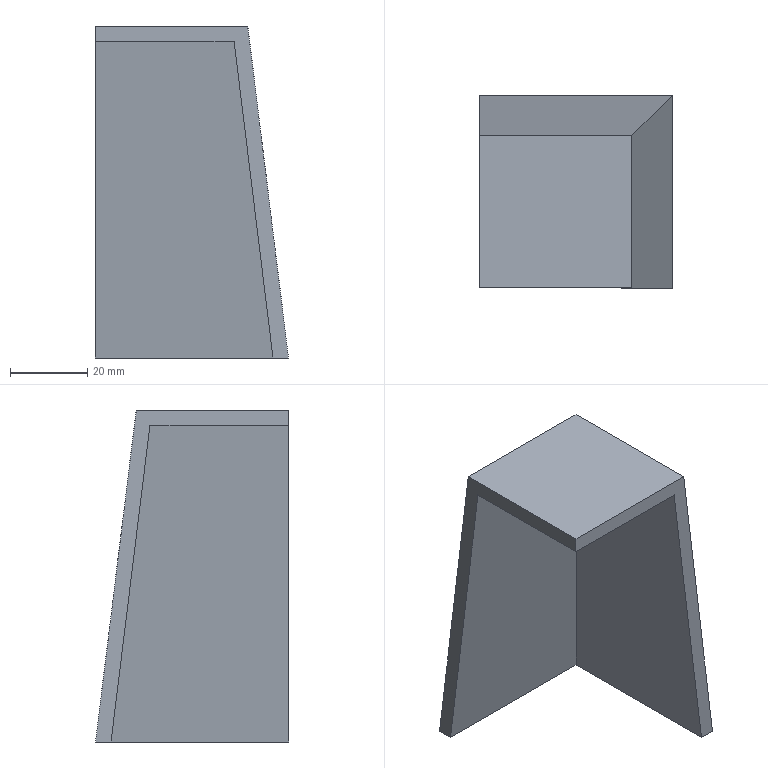Component | NX | STAND_2 | 1 solid | 9 faces | box 50 x 50 x 86 mm | volume 34687 mm3 | plane 9
STEP:
#1=CARTESIAN_POINT('',(0.,0.,0.));
#2=DIRECTION('',(0.,0.,1.));
#3=DIRECTION('',(1.,0.,0.));
#4=AXIS2_PLACEMENT_3D('',#1,#2,#3);
#5=CARTESIAN_POINT('',(223.059,445.97,-786.));
#6=VERTEX_POINT('',#5);
#7=CARTESIAN_POINT('',(223.059,450.,-786.));
#8=VERTEX_POINT('',#7);
#9=CARTESIAN_POINT('',(223.059,400.,-786.));
#10=DIRECTION('',(0.,1.,0.));
#11=VECTOR('',#10,1.);
#12=LINE('',#9,#11);
#13=CARTESIAN_POINT('',(223.059,400.,-770.));
#14=DIRECTION('',(-1.,0.,0.));
#15=DIRECTION('',(0.,0.,-1.));
#16=AXIS2_PLACEMENT_3D('',#13,#14,#15);
#17=PLANE('',#16);
#18=CARTESIAN_POINT('',(16.,0.));
#19=DIRECTION('',(0.,-1.));
#20=VECTOR('',#19,1.);
#21=LINE('',#18,#20);
#22=(GEOMETRIC_REPRESENTATION_CONTEXT(2)PARAMETRIC_REPRESENTATION_CONTEXT()REPRESENTATION_CONTEXT('',''));
#23=DEFINITIONAL_REPRESENTATION('',(#21),#22);
#24=PCURVE('',#17,#23);
#25=CARTESIAN_POINT('',(273.059,400.,-786.));
#26=DIRECTION('',(0.,0.,-1.));
#27=DIRECTION('',(1.,0.,0.));
#28=AXIS2_PLACEMENT_3D('',#25,#26,#27);
#29=PLANE('',#28);
#30=CARTESIAN_POINT('',(-50.,0.));
#31=DIRECTION('',(0.,-1.));
#32=VECTOR('',#31,1.);
#33=LINE('',#30,#32);
#34=(GEOMETRIC_REPRESENTATION_CONTEXT(2)PARAMETRIC_REPRESENTATION_CONTEXT()REPRESENTATION_CONTEXT('',''));
#35=DEFINITIONAL_REPRESENTATION('',(#33),#34);
#36=PCURVE('',#29,#35);
#37=SURFACE_CURVE('',#12,(#24,#36),.PCURVE_S1.);
#38=EDGE_CURVE('',#6,#8,#37,.T.);
#39=ORIENTED_EDGE('',*,*,#38,.F.);
#40=CARTESIAN_POINT('',(223.059,435.902,-704.));
#41=VERTEX_POINT('',#40);
#42=CARTESIAN_POINT('',(223.059,446.03,-786.487));
#43=DIRECTION('',(0.,-0.1219,0.9925));
#44=VECTOR('',#43,1.);
#45=LINE('',#42,#44);
#46=CARTESIAN_POINT('',(16.487,-46.03));
#47=DIRECTION('',(-0.9925,0.1219));
#48=VECTOR('',#47,1.);
#49=LINE('',#46,#48);
#50=(GEOMETRIC_REPRESENTATION_CONTEXT(2)PARAMETRIC_REPRESENTATION_CONTEXT()REPRESENTATION_CONTEXT('',''));
#51=DEFINITIONAL_REPRESENTATION('',(#49),#50);
#52=PCURVE('',#17,#51);
#53=CARTESIAN_POINT('',(248.059,446.03,-786.487));
#54=DIRECTION('',(0.,-0.9925,-0.1219));
#55=DIRECTION('',(0.,-0.1219,0.9925));
#56=AXIS2_PLACEMENT_3D('',#53,#54,#55);
#57=PLANE('',#56);
#58=CARTESIAN_POINT('',(0.,25.));
#59=DIRECTION('',(1.,0.));
#60=VECTOR('',#59,1.);
#61=LINE('',#58,#60);
#62=(GEOMETRIC_REPRESENTATION_CONTEXT(2)PARAMETRIC_REPRESENTATION_CONTEXT()REPRESENTATION_CONTEXT('',''));
#63=DEFINITIONAL_REPRESENTATION('',(#61),#62);
#64=PCURVE('',#57,#63);
#65=SURFACE_CURVE('',#45,(#52,#64),.PCURVE_S1.);
#66=EDGE_CURVE('',#6,#41,#65,.T.);
#67=ORIENTED_EDGE('',*,*,#66,.T.);
#68=CARTESIAN_POINT('',(223.059,400.,-704.));
#69=VERTEX_POINT('',#68);
#70=CARTESIAN_POINT('',(223.059,400.,-704.));
#71=DIRECTION('',(0.,1.,0.));
#72=VECTOR('',#71,1.);
#73=LINE('',#70,#72);
#74=CARTESIAN_POINT('',(-66.,0.));
#75=DIRECTION('',(0.,-1.));
#76=VECTOR('',#75,1.);
#77=LINE('',#74,#76);
#78=(GEOMETRIC_REPRESENTATION_CONTEXT(2)PARAMETRIC_REPRESENTATION_CONTEXT()REPRESENTATION_CONTEXT('',''));
#79=DEFINITIONAL_REPRESENTATION('',(#77),#78);
#80=PCURVE('',#17,#79);
#81=CARTESIAN_POINT('',(223.059,400.,-704.));
#82=DIRECTION('',(0.,0.,1.));
#83=DIRECTION('',(-1.,0.,0.));
#84=AXIS2_PLACEMENT_3D('',#81,#82,#83);
#85=PLANE('',#84);
#86=CARTESIAN_POINT('',(0.,0.));
#87=DIRECTION('',(0.,-1.));
#88=VECTOR('',#87,1.);
#89=LINE('',#86,#88);
#90=(GEOMETRIC_REPRESENTATION_CONTEXT(2)PARAMETRIC_REPRESENTATION_CONTEXT()REPRESENTATION_CONTEXT('',''));
#91=DEFINITIONAL_REPRESENTATION('',(#89),#90);
#92=PCURVE('',#85,#91);
#93=SURFACE_CURVE('',#73,(#80,#92),.PCURVE_S1.);
#94=EDGE_CURVE('',#69,#41,#93,.T.);
#95=ORIENTED_EDGE('',*,*,#94,.F.);
#96=CARTESIAN_POINT('',(223.059,400.,-700.));
#97=VERTEX_POINT('',#96);
#98=CARTESIAN_POINT('',(223.059,400.,-770.));
#99=DIRECTION('',(0.,0.,1.));
#100=VECTOR('',#99,1.);
#101=LINE('',#98,#100);
#102=CARTESIAN_POINT('',(0.,0.));
#103=DIRECTION('',(-1.,0.));
#104=VECTOR('',#103,1.);
#105=LINE('',#102,#104);
#106=(GEOMETRIC_REPRESENTATION_CONTEXT(2)PARAMETRIC_REPRESENTATION_CONTEXT()REPRESENTATION_CONTEXT('',''));
#107=DEFINITIONAL_REPRESENTATION('',(#105),#106);
#108=PCURVE('',#17,#107);
#109=CARTESIAN_POINT('',(0.,400.,0.));
#110=DIRECTION('',(0.,1.,0.));
#111=DIRECTION('',(0.,0.,-1.));
#112=AXIS2_PLACEMENT_3D('',#109,#110,#111);
#113=PLANE('',#112);
#114=CARTESIAN_POINT('',(770.,-223.059));
#115=DIRECTION('',(-1.,0.));
#116=VECTOR('',#115,1.);
#117=LINE('',#114,#116);
#118=(GEOMETRIC_REPRESENTATION_CONTEXT(2)PARAMETRIC_REPRESENTATION_CONTEXT()REPRESENTATION_CONTEXT('',''));
#119=DEFINITIONAL_REPRESENTATION('',(#117),#118);
#120=PCURVE('',#113,#119);
#121=SURFACE_CURVE('',#101,(#108,#120),.PCURVE_S1.);
#122=EDGE_CURVE('',#69,#97,#121,.T.);
#123=ORIENTED_EDGE('',*,*,#122,.T.);
#124=CARTESIAN_POINT('',(223.059,439.441,-700.));
#125=VERTEX_POINT('',#124);
#126=CARTESIAN_POINT('',(223.059,400.,-700.));
#127=DIRECTION('',(0.,1.,0.));
#128=VECTOR('',#127,1.);
#129=LINE('',#126,#128);
#130=CARTESIAN_POINT('',(-70.,0.));
#131=DIRECTION('',(0.,-1.));
#132=VECTOR('',#131,1.);
#133=LINE('',#130,#132);
#134=(GEOMETRIC_REPRESENTATION_CONTEXT(2)PARAMETRIC_REPRESENTATION_CONTEXT()REPRESENTATION_CONTEXT('',''));
#135=DEFINITIONAL_REPRESENTATION('',(#133),#134);
#136=PCURVE('',#17,#135);
#137=CARTESIAN_POINT('',(223.059,400.,-700.));
#138=DIRECTION('',(0.,0.,1.));
#139=DIRECTION('',(-1.,0.,0.));
#140=AXIS2_PLACEMENT_3D('',#137,#138,#139);
#141=PLANE('',#140);
#142=CARTESIAN_POINT('',(0.,0.));
#143=DIRECTION('',(0.,-1.));
#144=VECTOR('',#143,1.);
#145=LINE('',#142,#144);
#146=(GEOMETRIC_REPRESENTATION_CONTEXT(2)PARAMETRIC_REPRESENTATION_CONTEXT()REPRESENTATION_CONTEXT('',''));
#147=DEFINITIONAL_REPRESENTATION('',(#145),#146);
#148=PCURVE('',#141,#147);
#149=SURFACE_CURVE('',#129,(#136,#148),.PCURVE_S1.);
#150=EDGE_CURVE('',#97,#125,#149,.T.);
#151=ORIENTED_EDGE('',*,*,#150,.T.);
#152=CARTESIAN_POINT('',(223.059,450.,-786.));
#153=DIRECTION('',(0.,-0.1219,0.9925));
#154=VECTOR('',#153,1.);
#155=LINE('',#152,#154);
#156=CARTESIAN_POINT('',(16.,-50.));
#157=DIRECTION('',(-0.9925,0.1219));
#158=VECTOR('',#157,1.);
#159=LINE('',#156,#158);
#160=(GEOMETRIC_REPRESENTATION_CONTEXT(2)PARAMETRIC_REPRESENTATION_CONTEXT()REPRESENTATION_CONTEXT('',''));
#161=DEFINITIONAL_REPRESENTATION('',(#159),#160);
#162=PCURVE('',#17,#161);
#163=CARTESIAN_POINT('',(248.059,450.,-786.));
#164=DIRECTION('',(0.,-0.9925,-0.1219));
#165=DIRECTION('',(0.,-0.1219,0.9925));
#166=AXIS2_PLACEMENT_3D('',#163,#164,#165);
#167=PLANE('',#166);
#168=CARTESIAN_POINT('',(0.,25.));
#169=DIRECTION('',(1.,0.));
#170=VECTOR('',#169,1.);
#171=LINE('',#168,#170);
#172=(GEOMETRIC_REPRESENTATION_CONTEXT(2)PARAMETRIC_REPRESENTATION_CONTEXT()REPRESENTATION_CONTEXT('',''));
#173=DEFINITIONAL_REPRESENTATION('',(#171),#172);
#174=PCURVE('',#167,#173);
#175=SURFACE_CURVE('',#155,(#162,#174),.PCURVE_S1.);
#176=EDGE_CURVE('',#8,#125,#175,.T.);
#177=ORIENTED_EDGE('',*,*,#176,.F.);
#178=EDGE_LOOP('',(#39,#67,#95,#123,#151,#177));
#179=FACE_BOUND('',#178,.T.);
#180=ADVANCED_FACE('',(#179),#17,.T.);
#181=CARTESIAN_POINT('',(269.029,400.,-786.));
#182=VERTEX_POINT('',#181);
#183=CARTESIAN_POINT('',(269.029,445.97,-786.));
#184=VERTEX_POINT('',#183);
#185=CARTESIAN_POINT('',(269.029,425.,-786.));
#186=DIRECTION('',(0.,1.,0.));
#187=VECTOR('',#186,1.);
#188=LINE('',#185,#187);
#189=CARTESIAN_POINT('',(-4.03,-25.));
#190=DIRECTION('',(0.,-1.));
#191=VECTOR('',#190,1.);
#192=LINE('',#189,#191);
#193=(GEOMETRIC_REPRESENTATION_CONTEXT(2)PARAMETRIC_REPRESENTATION_CONTEXT()REPRESENTATION_CONTEXT('',''));
#194=DEFINITIONAL_REPRESENTATION('',(#192),#193);
#195=PCURVE('',#29,#194);
#196=CARTESIAN_POINT('',(269.089,425.,-786.487));
#197=DIRECTION('',(-0.9925,0.,-0.1219));
#198=DIRECTION('',(0.1219,0.,-0.9925));
#199=AXIS2_PLACEMENT_3D('',#196,#197,#198);
#200=PLANE('',#199);
#201=CARTESIAN_POINT('',(-0.4911,0.));
#202=DIRECTION('',(0.,-1.));
#203=VECTOR('',#202,1.);
#204=LINE('',#201,#203);
#205=(GEOMETRIC_REPRESENTATION_CONTEXT(2)PARAMETRIC_REPRESENTATION_CONTEXT()REPRESENTATION_CONTEXT('',''));
#206=DEFINITIONAL_REPRESENTATION('',(#204),#205);
#207=PCURVE('',#200,#206);
#208=SURFACE_CURVE('',#188,(#195,#207),.PCURVE_S1.);
#209=EDGE_CURVE('',#182,#184,#208,.T.);
#210=ORIENTED_EDGE('',*,*,#209,.T.);
#211=CARTESIAN_POINT('',(248.059,445.97,-786.));
#212=DIRECTION('',(-1.,0.,0.));
#213=VECTOR('',#212,1.);
#214=LINE('',#211,#213);
#215=CARTESIAN_POINT('',(-25.,-45.97));
#216=DIRECTION('',(-1.,0.));
#217=VECTOR('',#216,1.);
#218=LINE('',#215,#217);
#219=(GEOMETRIC_REPRESENTATION_CONTEXT(2)PARAMETRIC_REPRESENTATION_CONTEXT()REPRESENTATION_CONTEXT('',''));
#220=DEFINITIONAL_REPRESENTATION('',(#218),#219);
#221=PCURVE('',#29,#220);
#222=CARTESIAN_POINT('',(0.4911,0.));
#223=DIRECTION('',(0.,1.));
#224=VECTOR('',#223,1.);
#225=LINE('',#222,#224);
#226=(GEOMETRIC_REPRESENTATION_CONTEXT(2)PARAMETRIC_REPRESENTATION_CONTEXT()REPRESENTATION_CONTEXT('',''));
#227=DEFINITIONAL_REPRESENTATION('',(#225),#226);
#228=PCURVE('',#57,#227);
#229=SURFACE_CURVE('',#214,(#221,#228),.PCURVE_S1.);
#230=EDGE_CURVE('',#184,#6,#229,.T.);
#231=ORIENTED_EDGE('',*,*,#230,.T.);
#232=ORIENTED_EDGE('',*,*,#38,.T.);
#233=CARTESIAN_POINT('',(273.059,450.,-786.));
#234=VERTEX_POINT('',#233);
#235=CARTESIAN_POINT('',(248.059,450.,-786.));
#236=DIRECTION('',(-1.,0.,0.));
#237=VECTOR('',#236,1.);
#238=LINE('',#235,#237);
#239=CARTESIAN_POINT('',(-25.,-50.));
#240=DIRECTION('',(-1.,0.));
#241=VECTOR('',#240,1.);
#242=LINE('',#239,#241);
#243=(GEOMETRIC_REPRESENTATION_CONTEXT(2)PARAMETRIC_REPRESENTATION_CONTEXT()REPRESENTATION_CONTEXT('',''));
#244=DEFINITIONAL_REPRESENTATION('',(#242),#243);
#245=PCURVE('',#29,#244);
#246=CARTESIAN_POINT('',(0.,0.));
#247=DIRECTION('',(0.,1.));
#248=VECTOR('',#247,1.);
#249=LINE('',#246,#248);
#250=(GEOMETRIC_REPRESENTATION_CONTEXT(2)PARAMETRIC_REPRESENTATION_CONTEXT()REPRESENTATION_CONTEXT('',''));
#251=DEFINITIONAL_REPRESENTATION('',(#249),#250);
#252=PCURVE('',#167,#251);
#253=SURFACE_CURVE('',#238,(#245,#252),.PCURVE_S1.);
#254=EDGE_CURVE('',#234,#8,#253,.T.);
#255=ORIENTED_EDGE('',*,*,#254,.F.);
#256=CARTESIAN_POINT('',(273.059,400.,-786.));
#257=VERTEX_POINT('',#256);
#258=CARTESIAN_POINT('',(273.059,425.,-786.));
#259=DIRECTION('',(0.,1.,0.));
#260=VECTOR('',#259,1.);
#261=LINE('',#258,#260);
#262=CARTESIAN_POINT('',(0.,-25.));
#263=DIRECTION('',(0.,-1.));
#264=VECTOR('',#263,1.);
#265=LINE('',#262,#264);
#266=(GEOMETRIC_REPRESENTATION_CONTEXT(2)PARAMETRIC_REPRESENTATION_CONTEXT()REPRESENTATION_CONTEXT('',''));
#267=DEFINITIONAL_REPRESENTATION('',(#265),#266);
#268=PCURVE('',#29,#267);
#269=CARTESIAN_POINT('',(273.059,425.,-786.));
#270=DIRECTION('',(-0.9925,0.,-0.1219));
#271=DIRECTION('',(0.1219,0.,-0.9925));
#272=AXIS2_PLACEMENT_3D('',#269,#270,#271);
#273=PLANE('',#272);
#274=CARTESIAN_POINT('',(0.,0.));
#275=DIRECTION('',(0.,-1.));
#276=VECTOR('',#275,1.);
#277=LINE('',#274,#276);
#278=(GEOMETRIC_REPRESENTATION_CONTEXT(2)PARAMETRIC_REPRESENTATION_CONTEXT()REPRESENTATION_CONTEXT('',''));
#279=DEFINITIONAL_REPRESENTATION('',(#277),#278);
#280=PCURVE('',#273,#279);
#281=SURFACE_CURVE('',#261,(#268,#280),.PCURVE_S1.);
#282=EDGE_CURVE('',#257,#234,#281,.T.);
#283=ORIENTED_EDGE('',*,*,#282,.F.);
#284=CARTESIAN_POINT('',(273.059,400.,-786.));
#285=DIRECTION('',(-1.,0.,0.));
#286=VECTOR('',#285,1.);
#287=LINE('',#284,#286);
#288=CARTESIAN_POINT('',(0.,0.));
#289=DIRECTION('',(-1.,0.));
#290=VECTOR('',#289,1.);
#291=LINE('',#288,#290);
#292=(GEOMETRIC_REPRESENTATION_CONTEXT(2)PARAMETRIC_REPRESENTATION_CONTEXT()REPRESENTATION_CONTEXT('',''));
#293=DEFINITIONAL_REPRESENTATION('',(#291),#292);
#294=PCURVE('',#29,#293);
#295=CARTESIAN_POINT('',(786.,-273.059));
#296=DIRECTION('',(0.,1.));
#297=VECTOR('',#296,1.);
#298=LINE('',#295,#297);
#299=(GEOMETRIC_REPRESENTATION_CONTEXT(2)PARAMETRIC_REPRESENTATION_CONTEXT()REPRESENTATION_CONTEXT('',''));
#300=DEFINITIONAL_REPRESENTATION('',(#298),#299);
#301=PCURVE('',#113,#300);
#302=SURFACE_CURVE('',#287,(#294,#301),.PCURVE_S1.);
#303=EDGE_CURVE('',#257,#182,#302,.T.);
#304=ORIENTED_EDGE('',*,*,#303,.T.);
#305=EDGE_LOOP('',(#210,#231,#232,#255,#283,#304));
#306=FACE_BOUND('',#305,.T.);
#307=ADVANCED_FACE('',(#306),#29,.T.);
#308=CARTESIAN_POINT('',(262.499,439.441,-700.));
#309=VERTEX_POINT('',#308);
#310=CARTESIAN_POINT('',(248.059,439.441,-700.));
#311=DIRECTION('',(1.,0.,0.));
#312=VECTOR('',#311,1.);
#313=LINE('',#310,#312);
#314=CARTESIAN_POINT('',(-25.,-39.441));
#315=DIRECTION('',(-1.,0.));
#316=VECTOR('',#315,1.);
#317=LINE('',#314,#316);
#318=(GEOMETRIC_REPRESENTATION_CONTEXT(2)PARAMETRIC_REPRESENTATION_CONTEXT()REPRESENTATION_CONTEXT('',''));
#319=DEFINITIONAL_REPRESENTATION('',(#317),#318);
#320=PCURVE('',#141,#319);
#321=CARTESIAN_POINT('',(86.646,0.));
#322=DIRECTION('',(0.,-1.));
#323=VECTOR('',#322,1.);
#324=LINE('',#321,#323);
#325=(GEOMETRIC_REPRESENTATION_CONTEXT(2)PARAMETRIC_REPRESENTATION_CONTEXT()REPRESENTATION_CONTEXT('',''));
#326=DEFINITIONAL_REPRESENTATION('',(#324),#325);
#327=PCURVE('',#167,#326);
#328=SURFACE_CURVE('',#313,(#320,#327),.PCURVE_S1.);
#329=EDGE_CURVE('',#125,#309,#328,.T.);
#330=ORIENTED_EDGE('',*,*,#329,.F.);
#331=ORIENTED_EDGE('',*,*,#150,.F.);
#332=CARTESIAN_POINT('',(262.499,400.,-700.));
#333=VERTEX_POINT('',#332);
#334=CARTESIAN_POINT('',(223.059,400.,-700.));
#335=DIRECTION('',(1.,0.,0.));
#336=VECTOR('',#335,1.);
#337=LINE('',#334,#336);
#338=CARTESIAN_POINT('',(0.,0.));
#339=DIRECTION('',(-1.,0.));
#340=VECTOR('',#339,1.);
#341=LINE('',#338,#340);
#342=(GEOMETRIC_REPRESENTATION_CONTEXT(2)PARAMETRIC_REPRESENTATION_CONTEXT()REPRESENTATION_CONTEXT('',''));
#343=DEFINITIONAL_REPRESENTATION('',(#341),#342);
#344=PCURVE('',#141,#343);
#345=CARTESIAN_POINT('',(700.,-223.059));
#346=DIRECTION('',(0.,-1.));
#347=VECTOR('',#346,1.);
#348=LINE('',#345,#347);
#349=(GEOMETRIC_REPRESENTATION_CONTEXT(2)PARAMETRIC_REPRESENTATION_CONTEXT()REPRESENTATION_CONTEXT('',''));
#350=DEFINITIONAL_REPRESENTATION('',(#348),#349);
#351=PCURVE('',#113,#350);
#352=SURFACE_CURVE('',#337,(#344,#351),.PCURVE_S1.);
#353=EDGE_CURVE('',#97,#333,#352,.T.);
#354=ORIENTED_EDGE('',*,*,#353,.T.);
#355=CARTESIAN_POINT('',(262.499,400.,-700.));
#356=DIRECTION('',(0.,1.,0.));
#357=VECTOR('',#356,1.);
#358=LINE('',#355,#357);
#359=CARTESIAN_POINT('',(-39.441,0.));
#360=DIRECTION('',(0.,-1.));
#361=VECTOR('',#360,1.);
#362=LINE('',#359,#361);
#363=(GEOMETRIC_REPRESENTATION_CONTEXT(2)PARAMETRIC_REPRESENTATION_CONTEXT()REPRESENTATION_CONTEXT('',''));
#364=DEFINITIONAL_REPRESENTATION('',(#362),#363);
#365=PCURVE('',#141,#364);
#366=CARTESIAN_POINT('',(-86.646,25.));
#367=DIRECTION('',(0.,-1.));
#368=VECTOR('',#367,1.);
#369=LINE('',#366,#368);
#370=(GEOMETRIC_REPRESENTATION_CONTEXT(2)PARAMETRIC_REPRESENTATION_CONTEXT()REPRESENTATION_CONTEXT('',''));
#371=DEFINITIONAL_REPRESENTATION('',(#369),#370);
#372=PCURVE('',#273,#371);
#373=SURFACE_CURVE('',#358,(#365,#372),.PCURVE_S1.);
#374=EDGE_CURVE('',#333,#309,#373,.T.);
#375=ORIENTED_EDGE('',*,*,#374,.T.);
#376=EDGE_LOOP('',(#330,#331,#354,#375));
#377=FACE_BOUND('',#376,.T.);
#378=ADVANCED_FACE('',(#377),#141,.T.);
#379=CARTESIAN_POINT('',(272.693,449.634,-783.02));
#380=DIRECTION('',(0.121,0.121,-0.9853));
#381=VECTOR('',#380,1.);
#382=LINE('',#379,#381);
#383=CARTESIAN_POINT('',(-3.002,-24.634));
#384=DIRECTION('',(0.9927,-0.121));
#385=VECTOR('',#384,1.);
#386=LINE('',#383,#385);
#387=(GEOMETRIC_REPRESENTATION_CONTEXT(2)PARAMETRIC_REPRESENTATION_CONTEXT()REPRESENTATION_CONTEXT('',''));
#388=DEFINITIONAL_REPRESENTATION('',(#386),#387);
#389=PCURVE('',#273,#388);
#390=CARTESIAN_POINT('',(3.002,-24.634));
#391=DIRECTION('',(-0.9927,-0.121));
#392=VECTOR('',#391,1.);
#393=LINE('',#390,#392);
#394=(GEOMETRIC_REPRESENTATION_CONTEXT(2)PARAMETRIC_REPRESENTATION_CONTEXT()REPRESENTATION_CONTEXT('',''));
#395=DEFINITIONAL_REPRESENTATION('',(#393),#394);
#396=PCURVE('',#167,#395);
#397=SURFACE_CURVE('',#382,(#389,#396),.PCURVE_S1.);
#398=EDGE_CURVE('',#309,#234,#397,.T.);
#399=ORIENTED_EDGE('',*,*,#398,.F.);
#400=ORIENTED_EDGE('',*,*,#374,.F.);
#401=CARTESIAN_POINT('',(173.928,400.,21.356));
#402=DIRECTION('',(0.1219,0.,-0.9925));
#403=VECTOR('',#402,1.);
#404=LINE('',#401,#403);
#405=CARTESIAN_POINT('',(-813.419,25.));
#406=DIRECTION('',(1.,0.));
#407=VECTOR('',#406,1.);
#408=LINE('',#405,#407);
#409=(GEOMETRIC_REPRESENTATION_CONTEXT(2)PARAMETRIC_REPRESENTATION_CONTEXT()REPRESENTATION_CONTEXT('',''));
#410=DEFINITIONAL_REPRESENTATION('',(#408),#409);
#411=PCURVE('',#273,#410);
#412=CARTESIAN_POINT('',(-21.356,-173.928));
#413=DIRECTION('',(0.9925,-0.1219));
#414=VECTOR('',#413,1.);
#415=LINE('',#412,#414);
#416=(GEOMETRIC_REPRESENTATION_CONTEXT(2)PARAMETRIC_REPRESENTATION_CONTEXT()REPRESENTATION_CONTEXT('',''));
#417=DEFINITIONAL_REPRESENTATION('',(#415),#416);
#418=PCURVE('',#113,#417);
#419=SURFACE_CURVE('',#404,(#411,#418),.PCURVE_S1.);
#420=EDGE_CURVE('',#333,#257,#419,.T.);
#421=ORIENTED_EDGE('',*,*,#420,.T.);
#422=ORIENTED_EDGE('',*,*,#282,.T.);
#423=EDGE_LOOP('',(#399,#400,#421,#422));
#424=FACE_BOUND('',#423,.T.);
#425=ADVANCED_FACE('',(#424),#273,.F.);
#426=CARTESIAN_POINT('',(258.961,400.,-704.));
#427=VERTEX_POINT('',#426);
#428=CARTESIAN_POINT('',(0.,400.,-704.));
#429=DIRECTION('',(1.,0.,0.));
#430=VECTOR('',#429,1.);
#431=LINE('',#428,#430);
#432=CARTESIAN_POINT('',(704.,0.));
#433=DIRECTION('',(0.,-1.));
#434=VECTOR('',#433,1.);
#435=LINE('',#432,#434);
#436=(GEOMETRIC_REPRESENTATION_CONTEXT(2)PARAMETRIC_REPRESENTATION_CONTEXT()REPRESENTATION_CONTEXT('',''));
#437=DEFINITIONAL_REPRESENTATION('',(#435),#436);
#438=PCURVE('',#113,#437);
#439=CARTESIAN_POINT('',(223.059,0.));
#440=DIRECTION('',(-1.,0.));
#441=VECTOR('',#440,1.);
#442=LINE('',#439,#441);
#443=(GEOMETRIC_REPRESENTATION_CONTEXT(2)PARAMETRIC_REPRESENTATION_CONTEXT()REPRESENTATION_CONTEXT('',''));
#444=DEFINITIONAL_REPRESENTATION('',(#442),#443);
#445=PCURVE('',#85,#444);
#446=SURFACE_CURVE('',#431,(#438,#445),.PCURVE_S1.);
#447=EDGE_CURVE('',#69,#427,#446,.T.);
#448=ORIENTED_EDGE('',*,*,#447,.T.);
#449=CARTESIAN_POINT('',(169.958,400.,20.868));
#450=DIRECTION('',(0.1219,0.,-0.9925));
#451=VECTOR('',#450,1.);
#452=LINE('',#449,#451);
#453=CARTESIAN_POINT('',(-20.868,-169.958));
#454=DIRECTION('',(0.9925,-0.1219));
#455=VECTOR('',#454,1.);
#456=LINE('',#453,#455);
#457=(GEOMETRIC_REPRESENTATION_CONTEXT(2)PARAMETRIC_REPRESENTATION_CONTEXT()REPRESENTATION_CONTEXT('',''));
#458=DEFINITIONAL_REPRESENTATION('',(#456),#457);
#459=PCURVE('',#113,#458);
#460=CARTESIAN_POINT('',(-813.419,25.));
#461=DIRECTION('',(1.,0.));
#462=VECTOR('',#461,1.);
#463=LINE('',#460,#462);
#464=(GEOMETRIC_REPRESENTATION_CONTEXT(2)PARAMETRIC_REPRESENTATION_CONTEXT()REPRESENTATION_CONTEXT('',''));
#465=DEFINITIONAL_REPRESENTATION('',(#463),#464);
#466=PCURVE('',#200,#465);
#467=SURFACE_CURVE('',#452,(#459,#466),.PCURVE_S1.);
#468=EDGE_CURVE('',#427,#182,#467,.T.);
#469=ORIENTED_EDGE('',*,*,#468,.T.);
#470=ORIENTED_EDGE('',*,*,#303,.F.);
#471=ORIENTED_EDGE('',*,*,#420,.F.);
#472=ORIENTED_EDGE('',*,*,#353,.F.);
#473=ORIENTED_EDGE('',*,*,#122,.F.);
#474=EDGE_LOOP('',(#448,#469,#470,#471,#472,#473));
#475=FACE_BOUND('',#474,.T.);
#476=ADVANCED_FACE('',(#475),#113,.F.);
#477=ORIENTED_EDGE('',*,*,#176,.T.);
#478=ORIENTED_EDGE('',*,*,#329,.T.);
#479=ORIENTED_EDGE('',*,*,#398,.T.);
#480=ORIENTED_EDGE('',*,*,#254,.T.);
#481=EDGE_LOOP('',(#477,#478,#479,#480));
#482=FACE_BOUND('',#481,.T.);
#483=ADVANCED_FACE('',(#482),#167,.F.);
#484=CARTESIAN_POINT('',(258.961,435.902,-704.));
#485=VERTEX_POINT('',#484);
#486=CARTESIAN_POINT('',(248.059,435.902,-704.));
#487=DIRECTION('',(1.,0.,0.));
#488=VECTOR('',#487,1.);
#489=LINE('',#486,#488);
#490=CARTESIAN_POINT('',(-25.,-35.902));
#491=DIRECTION('',(-1.,0.));
#492=VECTOR('',#491,1.);
#493=LINE('',#490,#492);
#494=(GEOMETRIC_REPRESENTATION_CONTEXT(2)PARAMETRIC_REPRESENTATION_CONTEXT()REPRESENTATION_CONTEXT('',''));
#495=DEFINITIONAL_REPRESENTATION('',(#493),#494);
#496=PCURVE('',#85,#495);
#497=CARTESIAN_POINT('',(83.107,0.));
#498=DIRECTION('',(0.,-1.));
#499=VECTOR('',#498,1.);
#500=LINE('',#497,#499);
#501=(GEOMETRIC_REPRESENTATION_CONTEXT(2)PARAMETRIC_REPRESENTATION_CONTEXT()REPRESENTATION_CONTEXT('',''));
#502=DEFINITIONAL_REPRESENTATION('',(#500),#501);
#503=PCURVE('',#57,#502);
#504=SURFACE_CURVE('',#489,(#496,#503),.PCURVE_S1.);
#505=EDGE_CURVE('',#41,#485,#504,.T.);
#506=ORIENTED_EDGE('',*,*,#505,.T.);
#507=CARTESIAN_POINT('',(258.961,400.,-704.));
#508=DIRECTION('',(0.,1.,0.));
#509=VECTOR('',#508,1.);
#510=LINE('',#507,#509);
#511=CARTESIAN_POINT('',(-35.902,0.));
#512=DIRECTION('',(0.,-1.));
#513=VECTOR('',#512,1.);
#514=LINE('',#511,#513);
#515=(GEOMETRIC_REPRESENTATION_CONTEXT(2)PARAMETRIC_REPRESENTATION_CONTEXT()REPRESENTATION_CONTEXT('',''));
#516=DEFINITIONAL_REPRESENTATION('',(#514),#515);
#517=PCURVE('',#85,#516);
#518=CARTESIAN_POINT('',(-83.107,25.));
#519=DIRECTION('',(0.,-1.));
#520=VECTOR('',#519,1.);
#521=LINE('',#518,#520);
#522=(GEOMETRIC_REPRESENTATION_CONTEXT(2)PARAMETRIC_REPRESENTATION_CONTEXT()REPRESENTATION_CONTEXT('',''));
#523=DEFINITIONAL_REPRESENTATION('',(#521),#522);
#524=PCURVE('',#200,#523);
#525=SURFACE_CURVE('',#510,(#517,#524),.PCURVE_S1.);
#526=EDGE_CURVE('',#427,#485,#525,.T.);
#527=ORIENTED_EDGE('',*,*,#526,.F.);
#528=ORIENTED_EDGE('',*,*,#447,.F.);
#529=ORIENTED_EDGE('',*,*,#94,.T.);
#530=EDGE_LOOP('',(#506,#527,#528,#529));
#531=FACE_BOUND('',#530,.T.);
#532=ADVANCED_FACE('',(#531),#85,.F.);
#533=CARTESIAN_POINT('',(268.781,445.722,-783.981));
#534=DIRECTION('',(0.121,0.121,-0.9853));
#535=VECTOR('',#534,1.);
#536=LINE('',#533,#535);
#537=CARTESIAN_POINT('',(-2.525,-20.722));
#538=DIRECTION('',(0.9927,-0.121));
#539=VECTOR('',#538,1.);
#540=LINE('',#537,#539);
#541=(GEOMETRIC_REPRESENTATION_CONTEXT(2)PARAMETRIC_REPRESENTATION_CONTEXT()REPRESENTATION_CONTEXT('',''));
#542=DEFINITIONAL_REPRESENTATION('',(#540),#541);
#543=PCURVE('',#200,#542);
#544=CARTESIAN_POINT('',(2.525,-20.722));
#545=DIRECTION('',(-0.9927,-0.121));
#546=VECTOR('',#545,1.);
#547=LINE('',#544,#546);
#548=(GEOMETRIC_REPRESENTATION_CONTEXT(2)PARAMETRIC_REPRESENTATION_CONTEXT()REPRESENTATION_CONTEXT('',''));
#549=DEFINITIONAL_REPRESENTATION('',(#547),#548);
#550=PCURVE('',#57,#549);
#551=SURFACE_CURVE('',#536,(#543,#550),.PCURVE_S1.);
#552=EDGE_CURVE('',#485,#184,#551,.T.);
#553=ORIENTED_EDGE('',*,*,#552,.T.);
#554=ORIENTED_EDGE('',*,*,#209,.F.);
#555=ORIENTED_EDGE('',*,*,#468,.F.);
#556=ORIENTED_EDGE('',*,*,#526,.T.);
#557=EDGE_LOOP('',(#553,#554,#555,#556));
#558=FACE_BOUND('',#557,.T.);
#559=ADVANCED_FACE('',(#558),#200,.T.);
#560=ORIENTED_EDGE('',*,*,#66,.F.);
#561=ORIENTED_EDGE('',*,*,#230,.F.);
#562=ORIENTED_EDGE('',*,*,#552,.F.);
#563=ORIENTED_EDGE('',*,*,#505,.F.);
#564=EDGE_LOOP('',(#560,#561,#562,#563));
#565=FACE_BOUND('',#564,.T.);
#566=ADVANCED_FACE('',(#565),#57,.T.);
#567=CLOSED_SHELL('',(#180,#307,#378,#425,#476,#483,#532,#559,#566));
#568=MANIFOLD_SOLID_BREP('',#567);
#569=(LENGTH_UNIT()NAMED_UNIT(*)SI_UNIT(.MILLI.,.METRE.));
#570=UNCERTAINTY_MEASURE_WITH_UNIT(LENGTH_MEASURE(0.0000001),#569,'','');
#571=(NAMED_UNIT(*)PLANE_ANGLE_UNIT()SI_UNIT($,.RADIAN.));
#572=(NAMED_UNIT(*)SI_UNIT($,.STERADIAN.)SOLID_ANGLE_UNIT());
#573=(GEOMETRIC_REPRESENTATION_CONTEXT(3)GLOBAL_UNCERTAINTY_ASSIGNED_CONTEXT((#570))GLOBAL_UNIT_ASSIGNED_CONTEXT((#569,#571,#572))REPRESENTATION_CONTEXT('',''));
#574=ADVANCED_BREP_SHAPE_REPRESENTATION('',(#4,#568),#573);